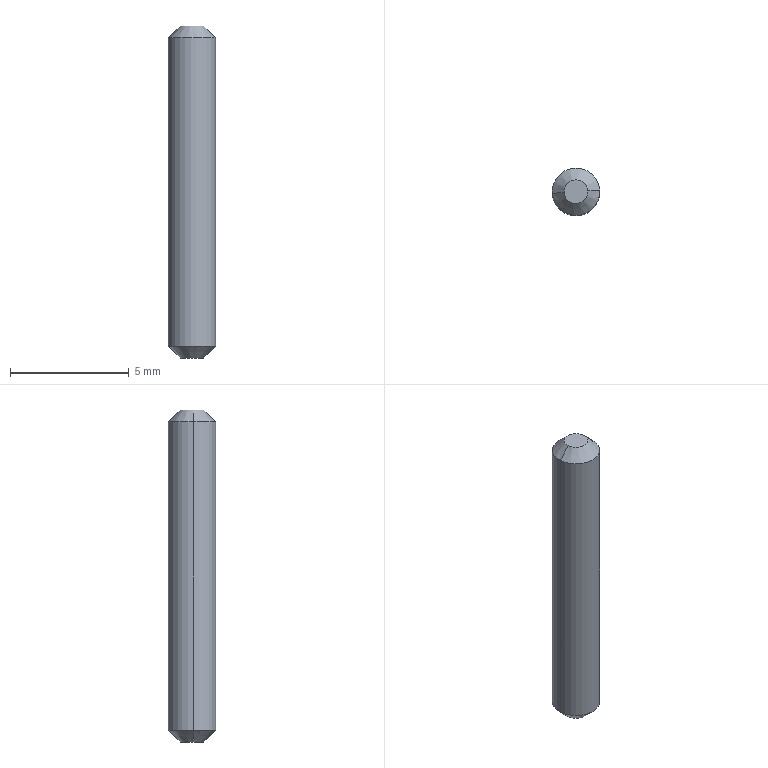Component | SolidWorks | MAC22-D2-L14-1 | 1 solid | 8 faces | box 2 x 2 x 14 mm | volume 43 mm3 | cone 4 | cylinder 2 | plane 2 | commonest cylinder face diameters 2 x2 | material Steel Part
STEP:
#1=COLOUR_RGB('',0.7922,0.8196,0.9333);
#2=FILL_AREA_STYLE_COLOUR('',#1);
#3=FILL_AREA_STYLE('',(#2));
#4=SURFACE_STYLE_FILL_AREA(#3);
#5=SURFACE_SIDE_STYLE('',(#4));
#6=SURFACE_STYLE_USAGE(.BOTH.,#5);
#7=PRESENTATION_STYLE_ASSIGNMENT((#6));
#8=CARTESIAN_POINT('',(-2.312,-0.8251,1.248));
#9=VERTEX_POINT('',#8);
#10=CARTESIAN_POINT('',(-2.234,-0.8196,1.248));
#11=VERTEX_POINT('',#10);
#12=CARTESIAN_POINT('',(-2.273,-0.8223,1.248));
#13=DIRECTION('',(0.,0.,1.));
#14=DIRECTION('',(-0.9976,-0.06964,0.));
#15=AXIS2_PLACEMENT_3D('',#12,#13,#14);
#16=CIRCLE('',#15,0.03937);
#17=EDGE_CURVE('',#9,#11,#16,.T.);
#18=ORIENTED_EDGE('',*,*,#17,.T.);
#19=CARTESIAN_POINT('',(-2.234,-0.8196,1.76));
#20=VERTEX_POINT('',#19);
#21=CARTESIAN_POINT('',(-2.234,-0.8196,1.229));
#22=DIRECTION('',(0.,0.,1.));
#23=VECTOR('',#22,39.37);
#24=LINE('',#21,#23);
#25=EDGE_CURVE('',#11,#20,#24,.T.);
#26=ORIENTED_EDGE('',*,*,#25,.T.);
#27=CARTESIAN_POINT('',(-2.312,-0.8251,1.76));
#28=VERTEX_POINT('',#27);
#29=CARTESIAN_POINT('',(-2.273,-0.8223,1.76));
#30=DIRECTION('',(0.,0.,-1.));
#31=DIRECTION('',(-0.9976,-0.06964,0.));
#32=AXIS2_PLACEMENT_3D('',#29,#30,#31);
#33=CIRCLE('',#32,0.03937);
#34=EDGE_CURVE('',#20,#28,#33,.T.);
#35=ORIENTED_EDGE('',*,*,#34,.T.);
#36=CARTESIAN_POINT('',(-2.312,-0.8251,1.229));
#37=DIRECTION('',(0.,0.,1.));
#38=VECTOR('',#37,39.37);
#39=LINE('',#36,#38);
#40=EDGE_CURVE('',#9,#28,#39,.T.);
#41=ORIENTED_EDGE('',*,*,#40,.F.);
#42=EDGE_LOOP('',(#18,#26,#35,#41));
#43=FACE_OUTER_BOUND('',#42,.T.);
#44=CARTESIAN_POINT('',(-2.273,-0.8223,1.229));
#45=DIRECTION('',(0.,0.,1.));
#46=DIRECTION('',(-0.9976,-0.06964,0.));
#47=AXIS2_PLACEMENT_3D('',#44,#45,#46);
#48=CYLINDRICAL_SURFACE('',#47,0.03937);
#49=ADVANCED_FACE('',(#43),#48,.T.);
#50=CARTESIAN_POINT('',(-2.254,-0.821,1.78));
#51=VERTEX_POINT('',#50);
#52=CARTESIAN_POINT('',(-2.293,-0.8237,1.78));
#53=VERTEX_POINT('',#52);
#54=CARTESIAN_POINT('',(-2.273,-0.8223,1.78));
#55=DIRECTION('',(0.,0.,-1.));
#56=DIRECTION('',(0.9976,0.06964,0.));
#57=AXIS2_PLACEMENT_3D('',#54,#55,#56);
#58=CIRCLE('',#57,0.01969);
#59=EDGE_CURVE('',#51,#53,#58,.T.);
#60=ORIENTED_EDGE('',*,*,#59,.T.);
#61=CARTESIAN_POINT('',(-2.312,-0.8251,1.76));
#62=DIRECTION('',(-0.7054,-0.04924,-0.7071));
#63=VECTOR('',#62,39.37);
#64=LINE('',#61,#63);
#65=EDGE_CURVE('',#53,#28,#64,.T.);
#66=ORIENTED_EDGE('',*,*,#65,.T.);
#67=ORIENTED_EDGE('',*,*,#34,.F.);
#68=CARTESIAN_POINT('',(-2.234,-0.8196,1.76));
#69=DIRECTION('',(0.7054,0.04924,-0.7071));
#70=VECTOR('',#69,39.37);
#71=LINE('',#68,#70);
#72=EDGE_CURVE('',#51,#20,#71,.T.);
#73=ORIENTED_EDGE('',*,*,#72,.F.);
#74=EDGE_LOOP('',(#60,#66,#67,#73));
#75=FACE_OUTER_BOUND('',#74,.T.);
#76=CARTESIAN_POINT('',(-2.273,-0.8223,1.76));
#77=DIRECTION('',(0.,0.,-1.));
#78=DIRECTION('',(0.9976,0.06964,0.));
#79=AXIS2_PLACEMENT_3D('',#76,#77,#78);
#80=CONICAL_SURFACE('',#79,0.03937,0.7854);
#81=ADVANCED_FACE('',(#75),#80,.T.);
#82=CARTESIAN_POINT('',(-2.293,-0.8237,1.229));
#83=VERTEX_POINT('',#82);
#84=CARTESIAN_POINT('',(-2.254,-0.821,1.229));
#85=VERTEX_POINT('',#84);
#86=CARTESIAN_POINT('',(-2.273,-0.8223,1.229));
#87=DIRECTION('',(0.,0.,1.));
#88=DIRECTION('',(-0.9976,-0.06964,0.));
#89=AXIS2_PLACEMENT_3D('',#86,#87,#88);
#90=CIRCLE('',#89,0.01969);
#91=EDGE_CURVE('',#83,#85,#90,.T.);
#92=ORIENTED_EDGE('',*,*,#91,.T.);
#93=CARTESIAN_POINT('',(-2.234,-0.8196,1.248));
#94=DIRECTION('',(0.7054,0.04924,0.7071));
#95=VECTOR('',#94,39.37);
#96=LINE('',#93,#95);
#97=EDGE_CURVE('',#85,#11,#96,.T.);
#98=ORIENTED_EDGE('',*,*,#97,.T.);
#99=ORIENTED_EDGE('',*,*,#17,.F.);
#100=CARTESIAN_POINT('',(-2.312,-0.8251,1.248));
#101=DIRECTION('',(-0.7054,-0.04924,0.7071));
#102=VECTOR('',#101,39.37);
#103=LINE('',#100,#102);
#104=EDGE_CURVE('',#83,#9,#103,.T.);
#105=ORIENTED_EDGE('',*,*,#104,.F.);
#106=EDGE_LOOP('',(#92,#98,#99,#105));
#107=FACE_OUTER_BOUND('',#106,.T.);
#108=CARTESIAN_POINT('',(-2.273,-0.8223,1.248));
#109=DIRECTION('',(0.,0.,1.));
#110=DIRECTION('',(-0.9976,-0.06964,0.));
#111=AXIS2_PLACEMENT_3D('',#108,#109,#110);
#112=CONICAL_SURFACE('',#111,0.03937,0.7854);
#113=ADVANCED_FACE('',(#107),#112,.T.);
#114=ORIENTED_EDGE('',*,*,#25,.F.);
#115=CARTESIAN_POINT('',(-2.273,-0.8223,1.248));
#116=DIRECTION('',(0.,0.,1.));
#117=DIRECTION('',(-0.9976,-0.06964,0.));
#118=AXIS2_PLACEMENT_3D('',#115,#116,#117);
#119=CIRCLE('',#118,0.03937);
#120=EDGE_CURVE('',#11,#9,#119,.T.);
#121=ORIENTED_EDGE('',*,*,#120,.T.);
#122=ORIENTED_EDGE('',*,*,#40,.T.);
#123=CARTESIAN_POINT('',(-2.273,-0.8223,1.76));
#124=DIRECTION('',(0.,0.,-1.));
#125=DIRECTION('',(-0.9976,-0.06964,0.));
#126=AXIS2_PLACEMENT_3D('',#123,#124,#125);
#127=CIRCLE('',#126,0.03937);
#128=EDGE_CURVE('',#28,#20,#127,.T.);
#129=ORIENTED_EDGE('',*,*,#128,.T.);
#130=EDGE_LOOP('',(#114,#121,#122,#129));
#131=FACE_OUTER_BOUND('',#130,.T.);
#132=CARTESIAN_POINT('',(-2.273,-0.8223,1.229));
#133=DIRECTION('',(0.,0.,1.));
#134=DIRECTION('',(-0.9976,-0.06964,0.));
#135=AXIS2_PLACEMENT_3D('',#132,#133,#134);
#136=CYLINDRICAL_SURFACE('',#135,0.03937);
#137=ADVANCED_FACE('',(#131),#136,.T.);
#138=ORIENTED_EDGE('',*,*,#65,.F.);
#139=CARTESIAN_POINT('',(-2.273,-0.8223,1.78));
#140=DIRECTION('',(0.,0.,-1.));
#141=DIRECTION('',(0.9976,0.06964,0.));
#142=AXIS2_PLACEMENT_3D('',#139,#140,#141);
#143=CIRCLE('',#142,0.01969);
#144=EDGE_CURVE('',#53,#51,#143,.T.);
#145=ORIENTED_EDGE('',*,*,#144,.T.);
#146=ORIENTED_EDGE('',*,*,#72,.T.);
#147=ORIENTED_EDGE('',*,*,#128,.F.);
#148=EDGE_LOOP('',(#138,#145,#146,#147));
#149=FACE_OUTER_BOUND('',#148,.T.);
#150=CARTESIAN_POINT('',(-2.273,-0.8223,1.76));
#151=DIRECTION('',(0.,0.,-1.));
#152=DIRECTION('',(0.9976,0.06964,0.));
#153=AXIS2_PLACEMENT_3D('',#150,#151,#152);
#154=CONICAL_SURFACE('',#153,0.03937,0.7854);
#155=ADVANCED_FACE('',(#149),#154,.T.);
#156=ORIENTED_EDGE('',*,*,#97,.F.);
#157=CARTESIAN_POINT('',(-2.273,-0.8223,1.229));
#158=DIRECTION('',(0.,0.,1.));
#159=DIRECTION('',(-0.9976,-0.06964,0.));
#160=AXIS2_PLACEMENT_3D('',#157,#158,#159);
#161=CIRCLE('',#160,0.01969);
#162=EDGE_CURVE('',#85,#83,#161,.T.);
#163=ORIENTED_EDGE('',*,*,#162,.T.);
#164=ORIENTED_EDGE('',*,*,#104,.T.);
#165=ORIENTED_EDGE('',*,*,#120,.F.);
#166=EDGE_LOOP('',(#156,#163,#164,#165));
#167=FACE_OUTER_BOUND('',#166,.T.);
#168=CARTESIAN_POINT('',(-2.273,-0.8223,1.248));
#169=DIRECTION('',(0.,0.,1.));
#170=DIRECTION('',(-0.9976,-0.06964,0.));
#171=AXIS2_PLACEMENT_3D('',#168,#169,#170);
#172=CONICAL_SURFACE('',#171,0.03937,0.7854);
#173=ADVANCED_FACE('',(#167),#172,.T.);
#174=ORIENTED_EDGE('',*,*,#59,.F.);
#175=ORIENTED_EDGE('',*,*,#144,.F.);
#176=EDGE_LOOP('',(#174,#175));
#177=FACE_OUTER_BOUND('',#176,.T.);
#178=CARTESIAN_POINT('',(-2.273,-0.8223,1.78));
#179=DIRECTION('',(0.,0.,-1.));
#180=DIRECTION('',(0.9976,0.06964,0.));
#181=AXIS2_PLACEMENT_3D('',#178,#179,#180);
#182=PLANE('',#181);
#183=ADVANCED_FACE('',(#177),#182,.F.);
#184=ORIENTED_EDGE('',*,*,#91,.F.);
#185=ORIENTED_EDGE('',*,*,#162,.F.);
#186=EDGE_LOOP('',(#184,#185));
#187=FACE_OUTER_BOUND('',#186,.T.);
#188=CARTESIAN_POINT('',(-2.272,-0.842,1.229));
#189=DIRECTION('',(0.,0.,1.));
#190=DIRECTION('',(-0.9976,-0.06964,0.));
#191=AXIS2_PLACEMENT_3D('',#188,#189,#190);
#192=PLANE('',#191);
#193=ADVANCED_FACE('',(#187),#192,.F.);
#194=CLOSED_SHELL('',(#49,#81,#113,#137,#155,#173,#183,#193));
#195=MANIFOLD_SOLID_BREP('',#194);
#196=STYLED_ITEM('',(#7),#195);
#197=(LENGTH_UNIT()NAMED_UNIT(*)SI_UNIT($,.METRE.));
#198=LENGTH_MEASURE_WITH_UNIT(LENGTH_MEASURE(0.0254),#197);
#199=DIMENSIONAL_EXPONENTS(1.,0.,0.,0.,0.,0.,0.);
#200=(CONVERSION_BASED_UNIT('',#198)LENGTH_UNIT()NAMED_UNIT(#199));
#201=UNCERTAINTY_MEASURE_WITH_UNIT(LENGTH_MEASURE(0.00001),#200,'','');
#202=(NAMED_UNIT(*)PLANE_ANGLE_UNIT()SI_UNIT($,.RADIAN.));
#203=(NAMED_UNIT(*)SI_UNIT($,.STERADIAN.)SOLID_ANGLE_UNIT());
#204=(GEOMETRIC_REPRESENTATION_CONTEXT(3)GLOBAL_UNCERTAINTY_ASSIGNED_CONTEXT((#201))GLOBAL_UNIT_ASSIGNED_CONTEXT((#200,#202,#203))REPRESENTATION_CONTEXT('',''));
#205=MECHANICAL_DESIGN_GEOMETRIC_PRESENTATION_REPRESENTATION('',(#196),#204);
#206=CARTESIAN_POINT('',(0.,0.,0.));
#207=DIRECTION('',(0.,0.,1.));
#208=DIRECTION('',(1.,0.,0.));
#209=AXIS2_PLACEMENT_3D('',#206,#207,#208);
#210=(LENGTH_UNIT()NAMED_UNIT(*)SI_UNIT($,.METRE.));
#211=LENGTH_MEASURE_WITH_UNIT(LENGTH_MEASURE(0.0254),#210);
#212=DIMENSIONAL_EXPONENTS(1.,0.,0.,0.,0.,0.,0.);
#213=(CONVERSION_BASED_UNIT('',#211)LENGTH_UNIT()NAMED_UNIT(#212));
#214=UNCERTAINTY_MEASURE_WITH_UNIT(LENGTH_MEASURE(0.00001),#213,'','');
#215=(NAMED_UNIT(*)PLANE_ANGLE_UNIT()SI_UNIT($,.RADIAN.));
#216=(NAMED_UNIT(*)SI_UNIT($,.STERADIAN.)SOLID_ANGLE_UNIT());
#217=(GEOMETRIC_REPRESENTATION_CONTEXT(3)GLOBAL_UNCERTAINTY_ASSIGNED_CONTEXT((#214))GLOBAL_UNIT_ASSIGNED_CONTEXT((#213,#215,#216))REPRESENTATION_CONTEXT('',''));
#218=ADVANCED_BREP_SHAPE_REPRESENTATION('',(#195,#209),#217);
#219=PRESENTATION_LAYER_ASSIGNMENT('','',(#196));